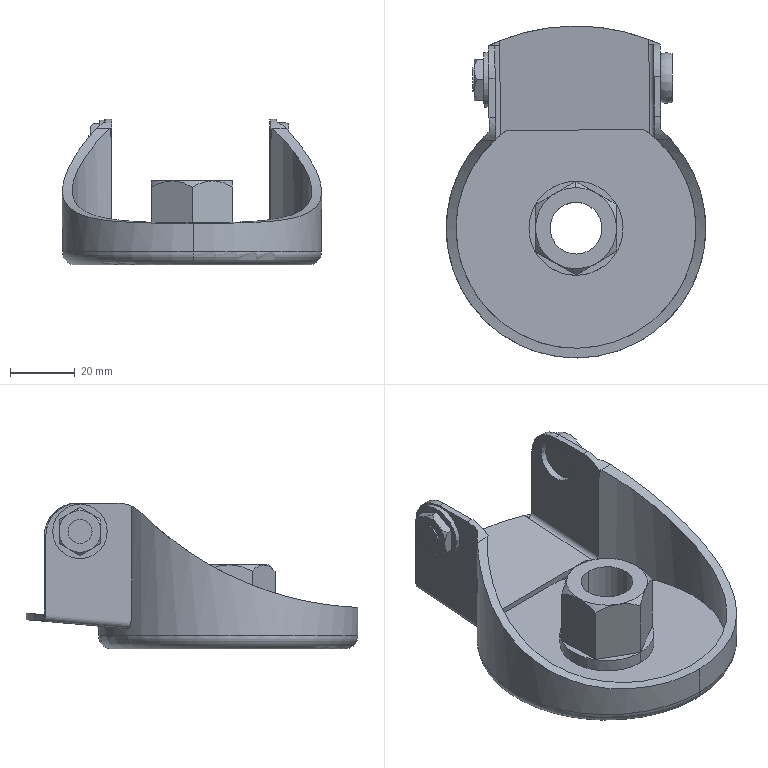Component | SolidWorks | CMAS50_F-2_CMAS50_Fbody-1 | 1 solid | 84 faces | box 80 x 102.36 x 44.92 mm | volume 38810 mm3 | plane 40 | cylinder 27 | cone 13 | torus 4 | commonest cylinder face diameters 13 x4 20 x4 16 x2 7.4 x2 16.8 x2 29 x2 80 x2 125.718 x2 | material 45
build123d program:
from build123d import *

# Parameters (mm, degrees)
SKETCH2_R                       = 8
EXTRUDE1_DEPTH                  = 16
EXTRUDE2_DEPTH                  = 40
EXTRUDE3_DEPTH                  = 50
EXTRUDE3_DEPTH_BACK             = 50
EXTRUDE4_DEPTH                  = 74
EXTRUDE5_DEPTH                  = 42
EXTRUDE6_DEPTH                  = 45
EXTRUDE6_DEPTH_BACK             = 45
SKETCH7_R                       = 6.5
SKETCH10_R                      = 20
EXTRUDE7_DEPTH                  = 37
SKETCH13_R                      = 9.25
EXTRUDE8_DEPTH                  = 5
SKETCH14_R                      = 8
M16_THREAD_MAJOR_DIA_BORE_DEPTH = 40


with BuildPart() as part:
    # Sketch1 → Revolve1 (revolve)
    with BuildSketch(Plane.XY, mode=Mode.PRIVATE) as revolve1_sk:
        with BuildLine():
            Line((0, -12.8), (36, -12.8))
            ThreePointArc((36, -12.8), (38.828, -13.972), (40, -16.8))
            Line((40, -16.8), (40, -56.8))
            Line((40, -56.8), (37, -56.8))
            Line((37, -56.8), (37, -15.3))
            Line((37, -15.3), (0, -15.3))
            Line((0, -15.3), (0, -12.8))
        make_face()
    revolve(revolve1_sk.sketch.rotate(Axis((0, -56.8, 0), (0, 1, 0)), 270), axis=Axis((0, -56.8, 0), (0, 1, 0)))

    # Sketch2 → Extrude1 (cut)
    with BuildSketch(Plane(origin=(0, 0, 0), x_dir=(1, 0, 0), z_dir=(0, 1, 0))):
        with Locations(Location((0, 0, 0), (0, 0, 270))):
            Circle(SKETCH2_R)
    extrude(amount=-EXTRUDE1_DEPTH, mode=Mode.SUBTRACT)

    # Sketch3 → Extrude2 (add)
    with BuildSketch(Plane(origin=(0, -2.789, 31.878), x_dir=(1, 0, 0), z_dir=(0, -0.08716, 0.9962))):
        with BuildLine():
            Line((-26.5, -18.28), (-26.5, -56.98))
            Line((-26.5, -56.98), (26.5, -56.98))
            Line((26.5, -56.98), (26.5, -18.28))
            ThreePointArc((26.5, -18.28), (25.914, -16.866), (24.5, -16.28))
            Line((24.5, -16.28), (-24.5, -16.28))
            ThreePointArc((-24.5, -16.28), (-25.914, -16.866), (-26.5, -18.28))
        make_face()
    extrude(amount=EXTRUDE2_DEPTH)

    # Sketch4 → Extrude3 (cut, two sides: drawn at the far end of the back side and taken through both)
    with BuildSketch(Plane(origin=(0, 0, 0), x_dir=(0, 0, -1), z_dir=(1, 0, 0)).offset(-EXTRUDE3_DEPTH_BACK)):
        with BuildLine():
            Line((-75, -24.912), (-75, -70))
            Line((-75, -70), (40, -70))
            Line((40, -70), (40, -25.6))
            ThreePointArc((40, -25.6), (3.636, -33.823), (-27.188, -54.794))
            ThreePointArc((-27.188, -54.794), (-30.431, -56.96), (-34.256, -57.72))
            Line((-34.256, -57.72), (-46.5, -57.72))
            ThreePointArc((-46.5, -57.72), (-53.571, -54.791), (-56.5, -47.72))
            Line((-56.5, -47.72), (-56.5, -23.293))
            Line((-56.5, -23.293), (-75, -24.912))
        make_face()
    extrude(amount=EXTRUDE3_DEPTH + EXTRUDE3_DEPTH_BACK, mode=Mode.SUBTRACT)

    # Sketch5 → Extrude4 (cut)
    with BuildSketch(Plane(origin=(0, 0, 0), x_dir=(1, 0, 0), z_dir=(0, 1, 0))):
        with BuildLine():
            Line((-26.5, -100), (26.5, -100))
            Line((26.5, -100), (26.5, -56.5))
            ThreePointArc((26.5, -56.5), (0, -62.359), (-26.5, -56.5))
            Line((-26.5, -56.5), (-26.5, -100))
        make_face()
    extrude(amount=-EXTRUDE4_DEPTH, mode=Mode.SUBTRACT)

    # Sketch6 → Extrude5 (cut)
    with BuildSketch(Plane(origin=(0, -2.353, 26.897), x_dir=(1, 0, 0), z_dir=(0, -0.08716, 0.9962))):
        with BuildLine():
            Line((-24.5, -19.78), (-24.5, -58.98))
            Line((-24.5, -58.98), (24.5, -58.98))
            Line((24.5, -58.98), (24.5, -19.78))
            ThreePointArc((24.5, -19.78), (24.061, -18.719), (23, -18.28))
            Line((23, -18.28), (-23, -18.28))
            ThreePointArc((-23, -18.28), (-24.061, -18.719), (-24.5, -19.78))
        make_face()
    extrude(amount=EXTRUDE5_DEPTH, mode=Mode.SUBTRACT)

    # Sketch7 → Extrude6 (cut, two sides: drawn at the far end of the back side and taken through both)
    with BuildSketch(Plane(origin=(0, 0, 0), x_dir=(0, 0, -1), z_dir=(1, 0, 0)).offset(-EXTRUDE6_DEPTH_BACK)):
        with Locations((-46, -49)):
            Circle(SKETCH7_R)
    extrude(amount=EXTRUDE6_DEPTH + EXTRUDE6_DEPTH_BACK, mode=Mode.SUBTRACT)

    # Sketch8 → Revolve2 (revolve)
    with BuildSketch(Plane(origin=(0, 0, 0), x_dir=(0, 0, -1), z_dir=(1, 0, 0)), mode=Mode.PRIVATE) as revolve2_sk:
        Polygon((0, -12.8), (14.5, -12.8), (14.5, -36.7), (12.5, -38.7), (0, -38.7), align=None)
    revolve(revolve2_sk.sketch.rotate(Axis((0, -38.7, 0), (0, 1, 0)), 180), axis=Axis((0, -38.7, 0), (0, 1, 0)))

    # Sketch9 → Cut-Revolve1 (revolve, cut)
    with BuildSketch(Plane(origin=(0, 0, 0), x_dir=(0, 0, -1), z_dir=(1, 0, 0)), mode=Mode.PRIVATE) as cut_revolve1_sk:
        Polygon((0, -12.8), (8, -12.8), (6.918, -13.883), (6.918, -37.617), (8, -38.7), (0, -38.7), align=None)
    revolve(cut_revolve1_sk.sketch.rotate(Axis((0, -38.7, 0), (0, 1, 0)), 180), axis=Axis((0, -38.7, 0), (0, 1, 0)), mode=Mode.SUBTRACT)

    # Sketch10 → Extrude7 (cut)
    with BuildSketch(Plane(origin=(0, -19.2, 0), x_dir=(1, 0, 0), z_dir=(0, 1, 0))):
        Circle(SKETCH10_R)
        Polygon((12.5, -7.217), (12.5, 7.217), (0, 14.434), (-12.5, 7.217), (-12.5, -7.217), (0, -14.434), align=None, mode=Mode.SUBTRACT)
    extrude(amount=-EXTRUDE7_DEPTH, mode=Mode.SUBTRACT)

    # Sketch11 → Revolve3 (revolve)
    with BuildSketch(Plane.XY.offset(46), mode=Mode.PRIVATE) as revolve3_sk:
        with BuildLine():
            Line((26.5, -49), (26.5, -41.6))
            ThreePointArc((26.5, -41.6), (28.35, -41.232), (30.2, -41.6))
            Line((30.2, -41.6), (30.2, -49))
            Line((30.2, -49), (26.5, -49))
        make_face()
    revolve(revolve3_sk.sketch.rotate(Axis((30.2, -49, 46), (-1, 0, 0)), 270), axis=Axis((30.2, -49, 46), (-1, 0, 0)))

    # Sketch12 → Revolve4 (revolve)
    with BuildSketch(Plane.XY.offset(46), mode=Mode.PRIVATE) as revolve4_sk:
        Polygon((-31.44, -49), (-31.44, -45.3), (-30.94, -45.3), (-30.94, -42.562), (-29.978, -41.6), (-28, -41.6), (-28, -40.6), (-26.5, -40.6), (-26.5, -49), align=None)
    revolve(revolve4_sk.sketch.rotate(Axis((-26.5, -49, 46), (-1, 0, 0)), 270), axis=Axis((-26.5, -49, 46), (-1, 0, 0)))

    # Sketch13 → Extrude8 (cut)
    with BuildSketch(Plane(origin=(-28, 0, 0), x_dir=(0, 0, -1), z_dir=(1, 0, 0))):
        with Locations((-46, -49)):
            Circle(SKETCH13_R)
        Polygon((-52.401, -45.304), (-52.401, -52.696), (-46, -56.391), (-39.599, -52.696), (-39.599, -45.304), (-46, -41.609), align=None, mode=Mode.SUBTRACT)
    extrude(amount=-EXTRUDE8_DEPTH, mode=Mode.SUBTRACT)

    # Sketch14 → M16 thread major-dia bore (cut, symmetric)
    with BuildSketch(Plane(origin=(0, 0, 0), x_dir=(1, 0, 0), z_dir=(0, 1, 0))):
        with Locations(Location((0, 0, 0), (0, 0, 270))):
            Circle(SKETCH14_R)
    extrude(amount=M16_THREAD_MAJOR_DIA_BORE_DEPTH, both=True, mode=Mode.SUBTRACT)


solid = part.part

# Placed as in the assembly
solid = solid.moved(Location((263.997, 558.998, 620.001), (-90.001, -0.544, 0.002949)))